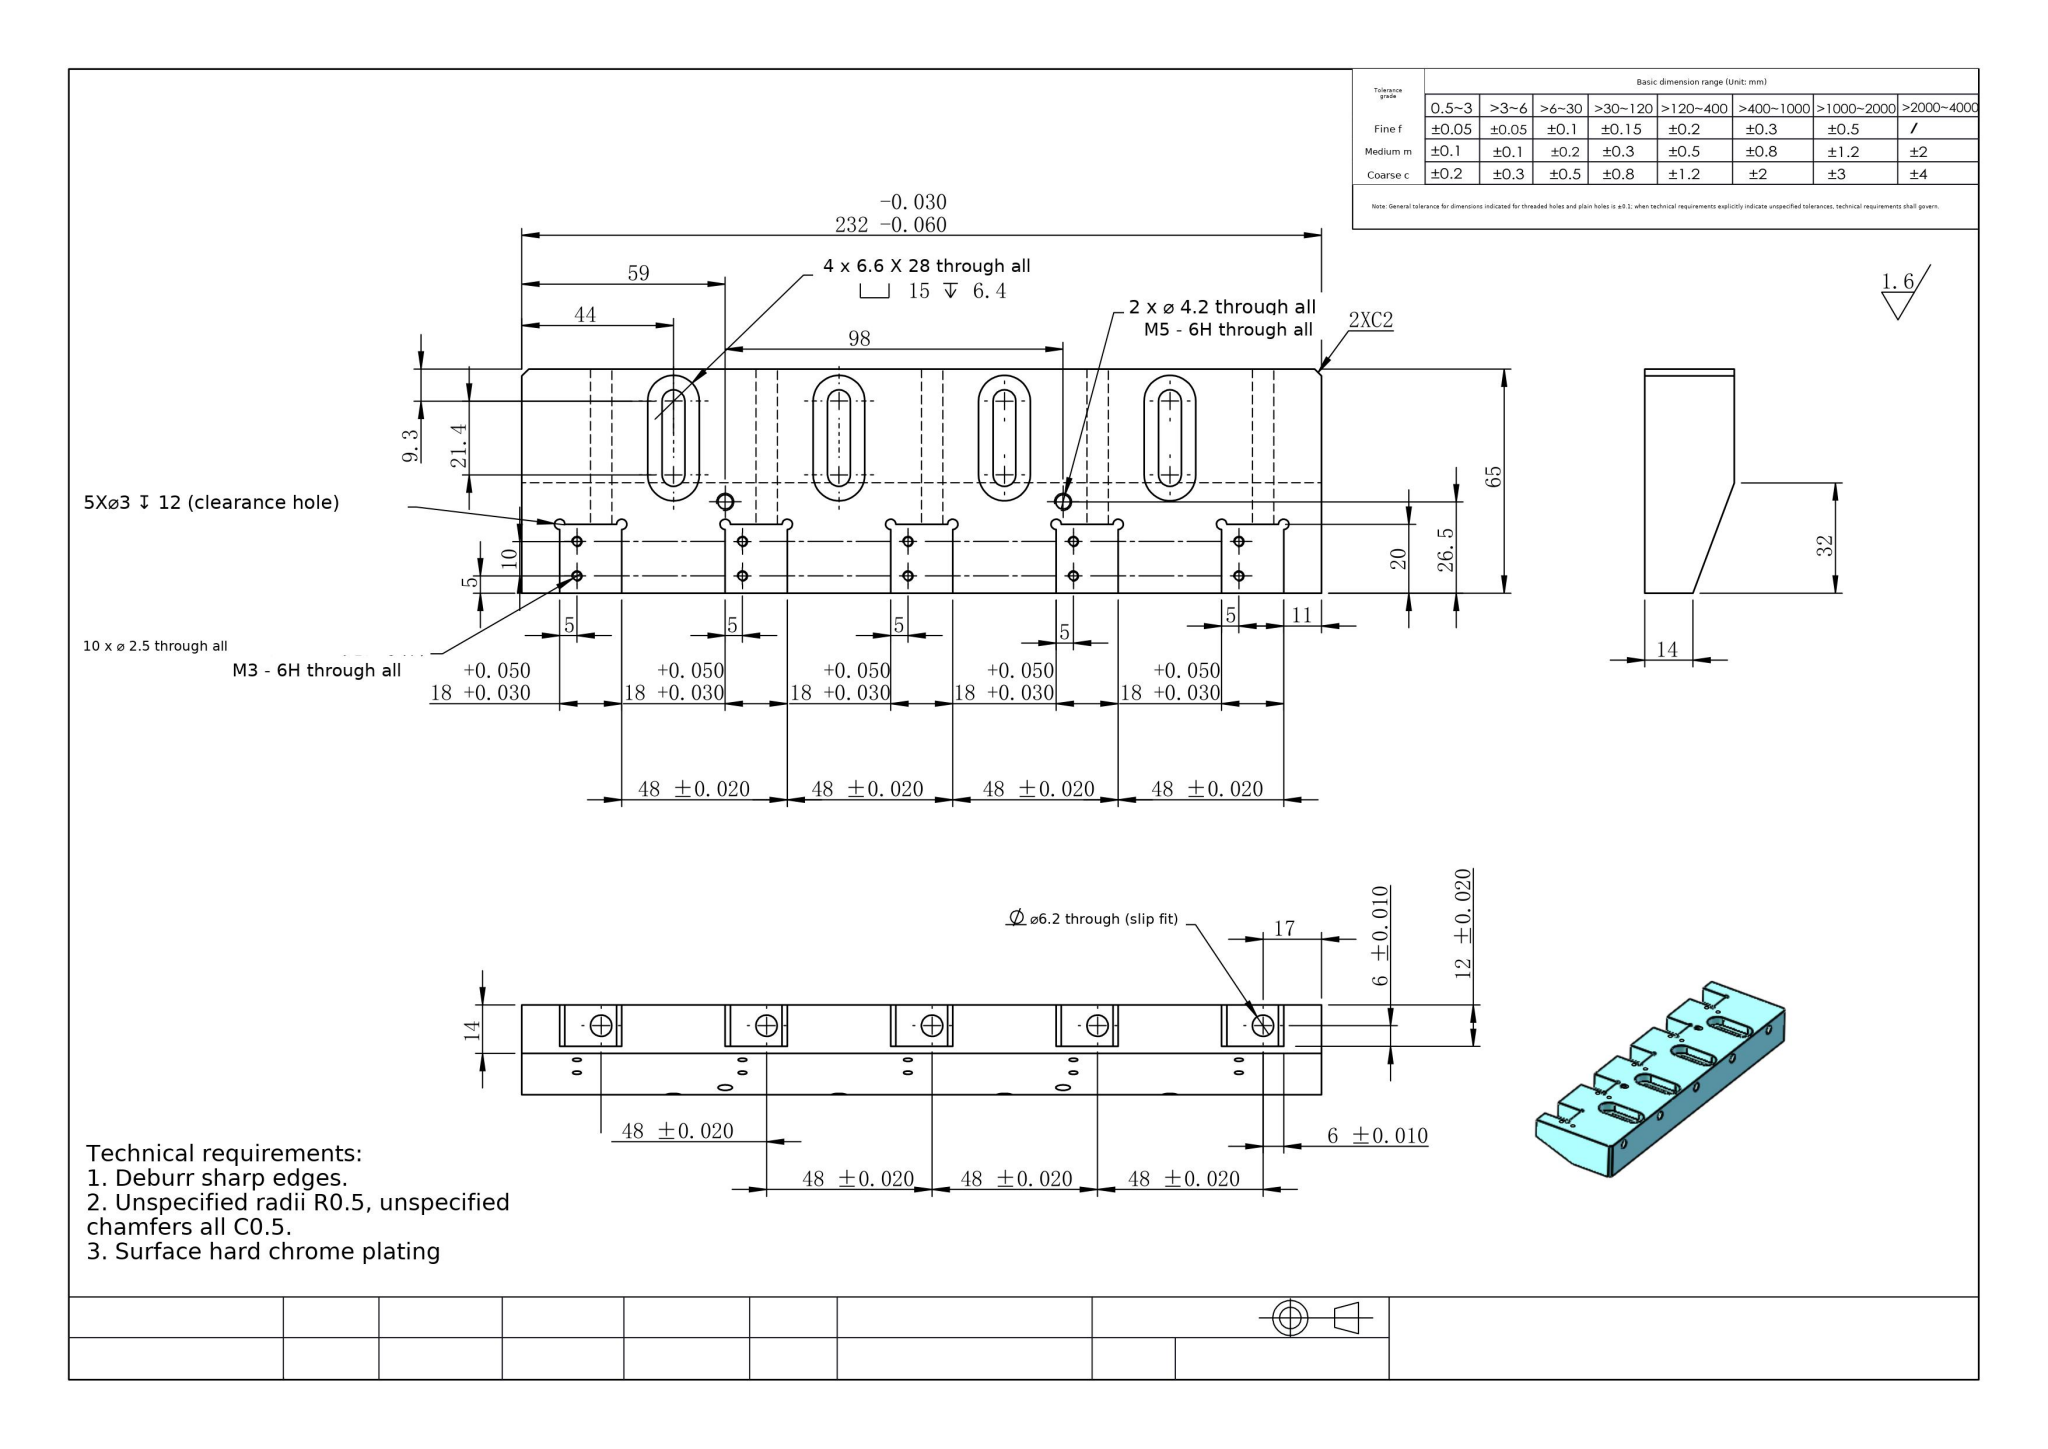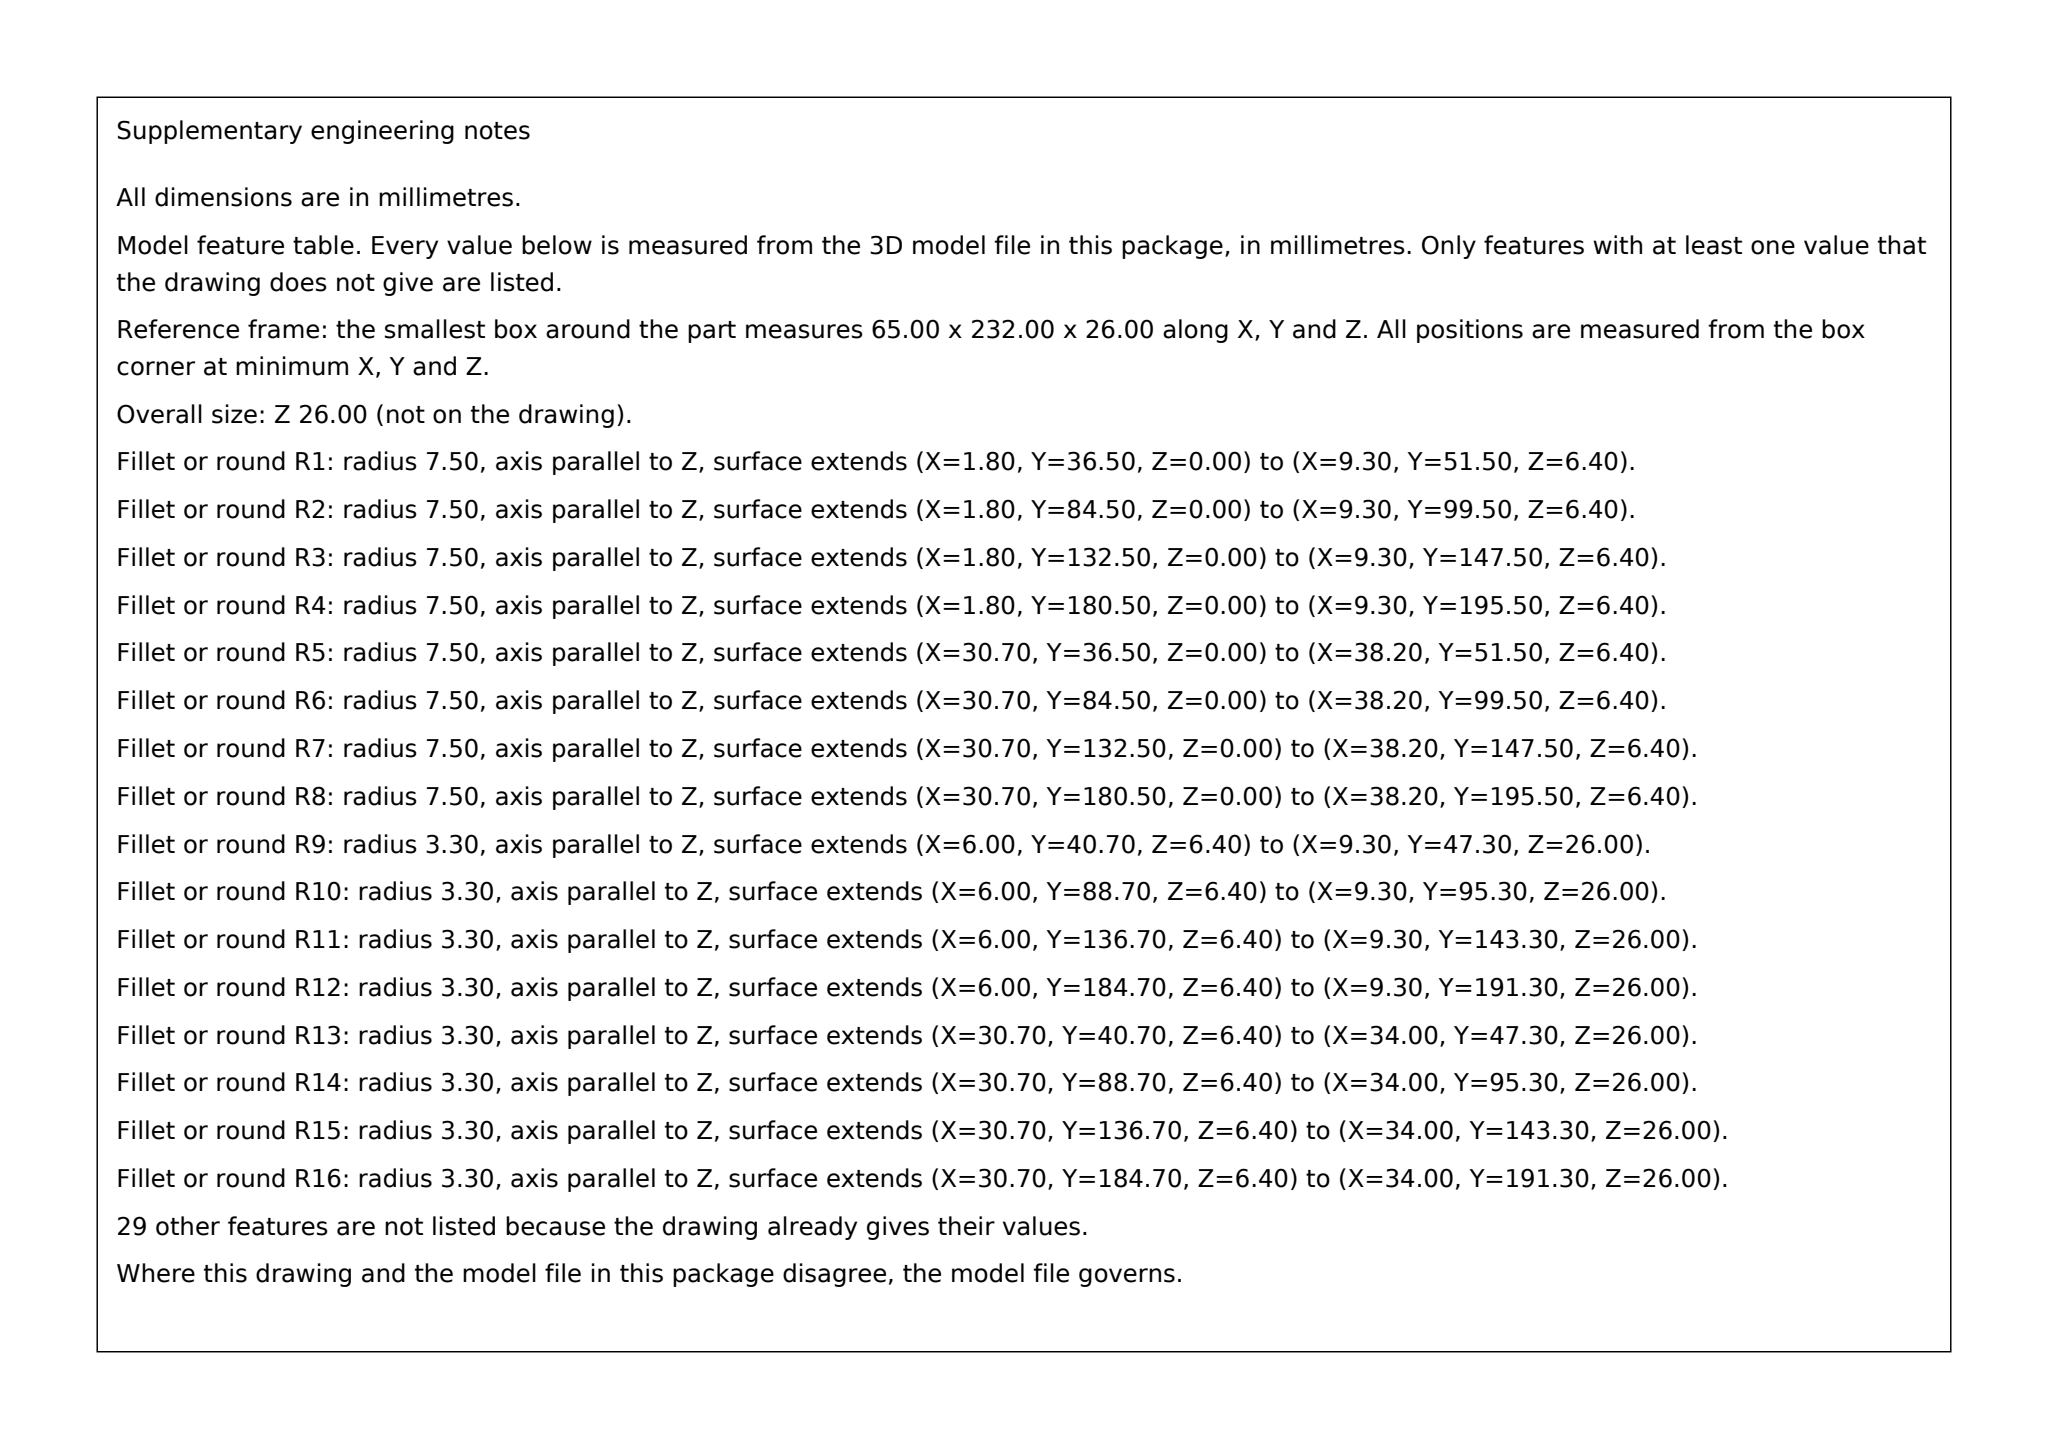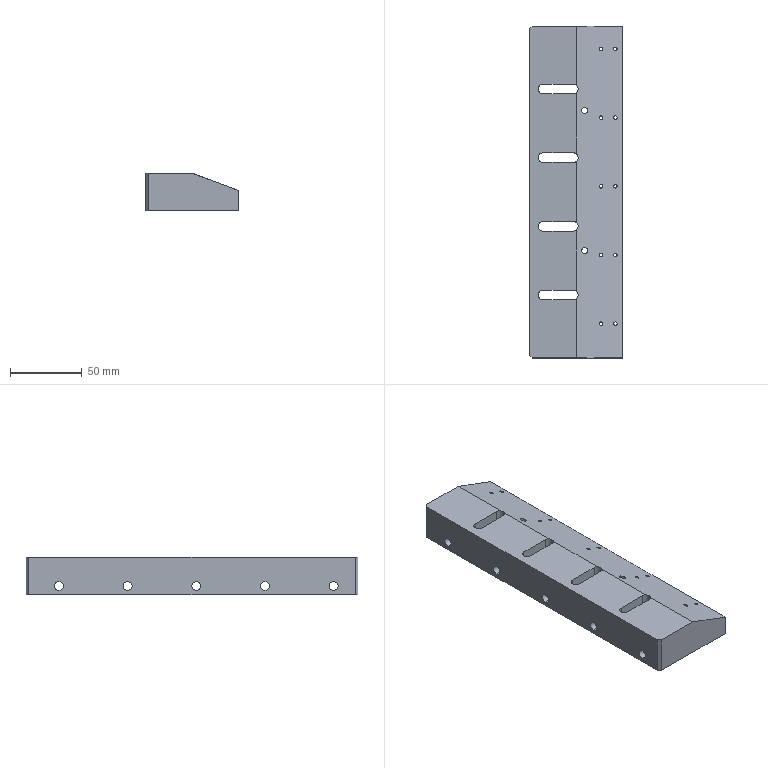Part | SolidWorks | mm | 1 solid | 127 faces | box 65 x 232 x 26 mm | volume 290962 mm3 | cylinder 78 | plane 49 | commonest cylinder face diameters 2.5 x20 3 x20 15 x12 6.6 x12 6.2 x10 4.2 x4